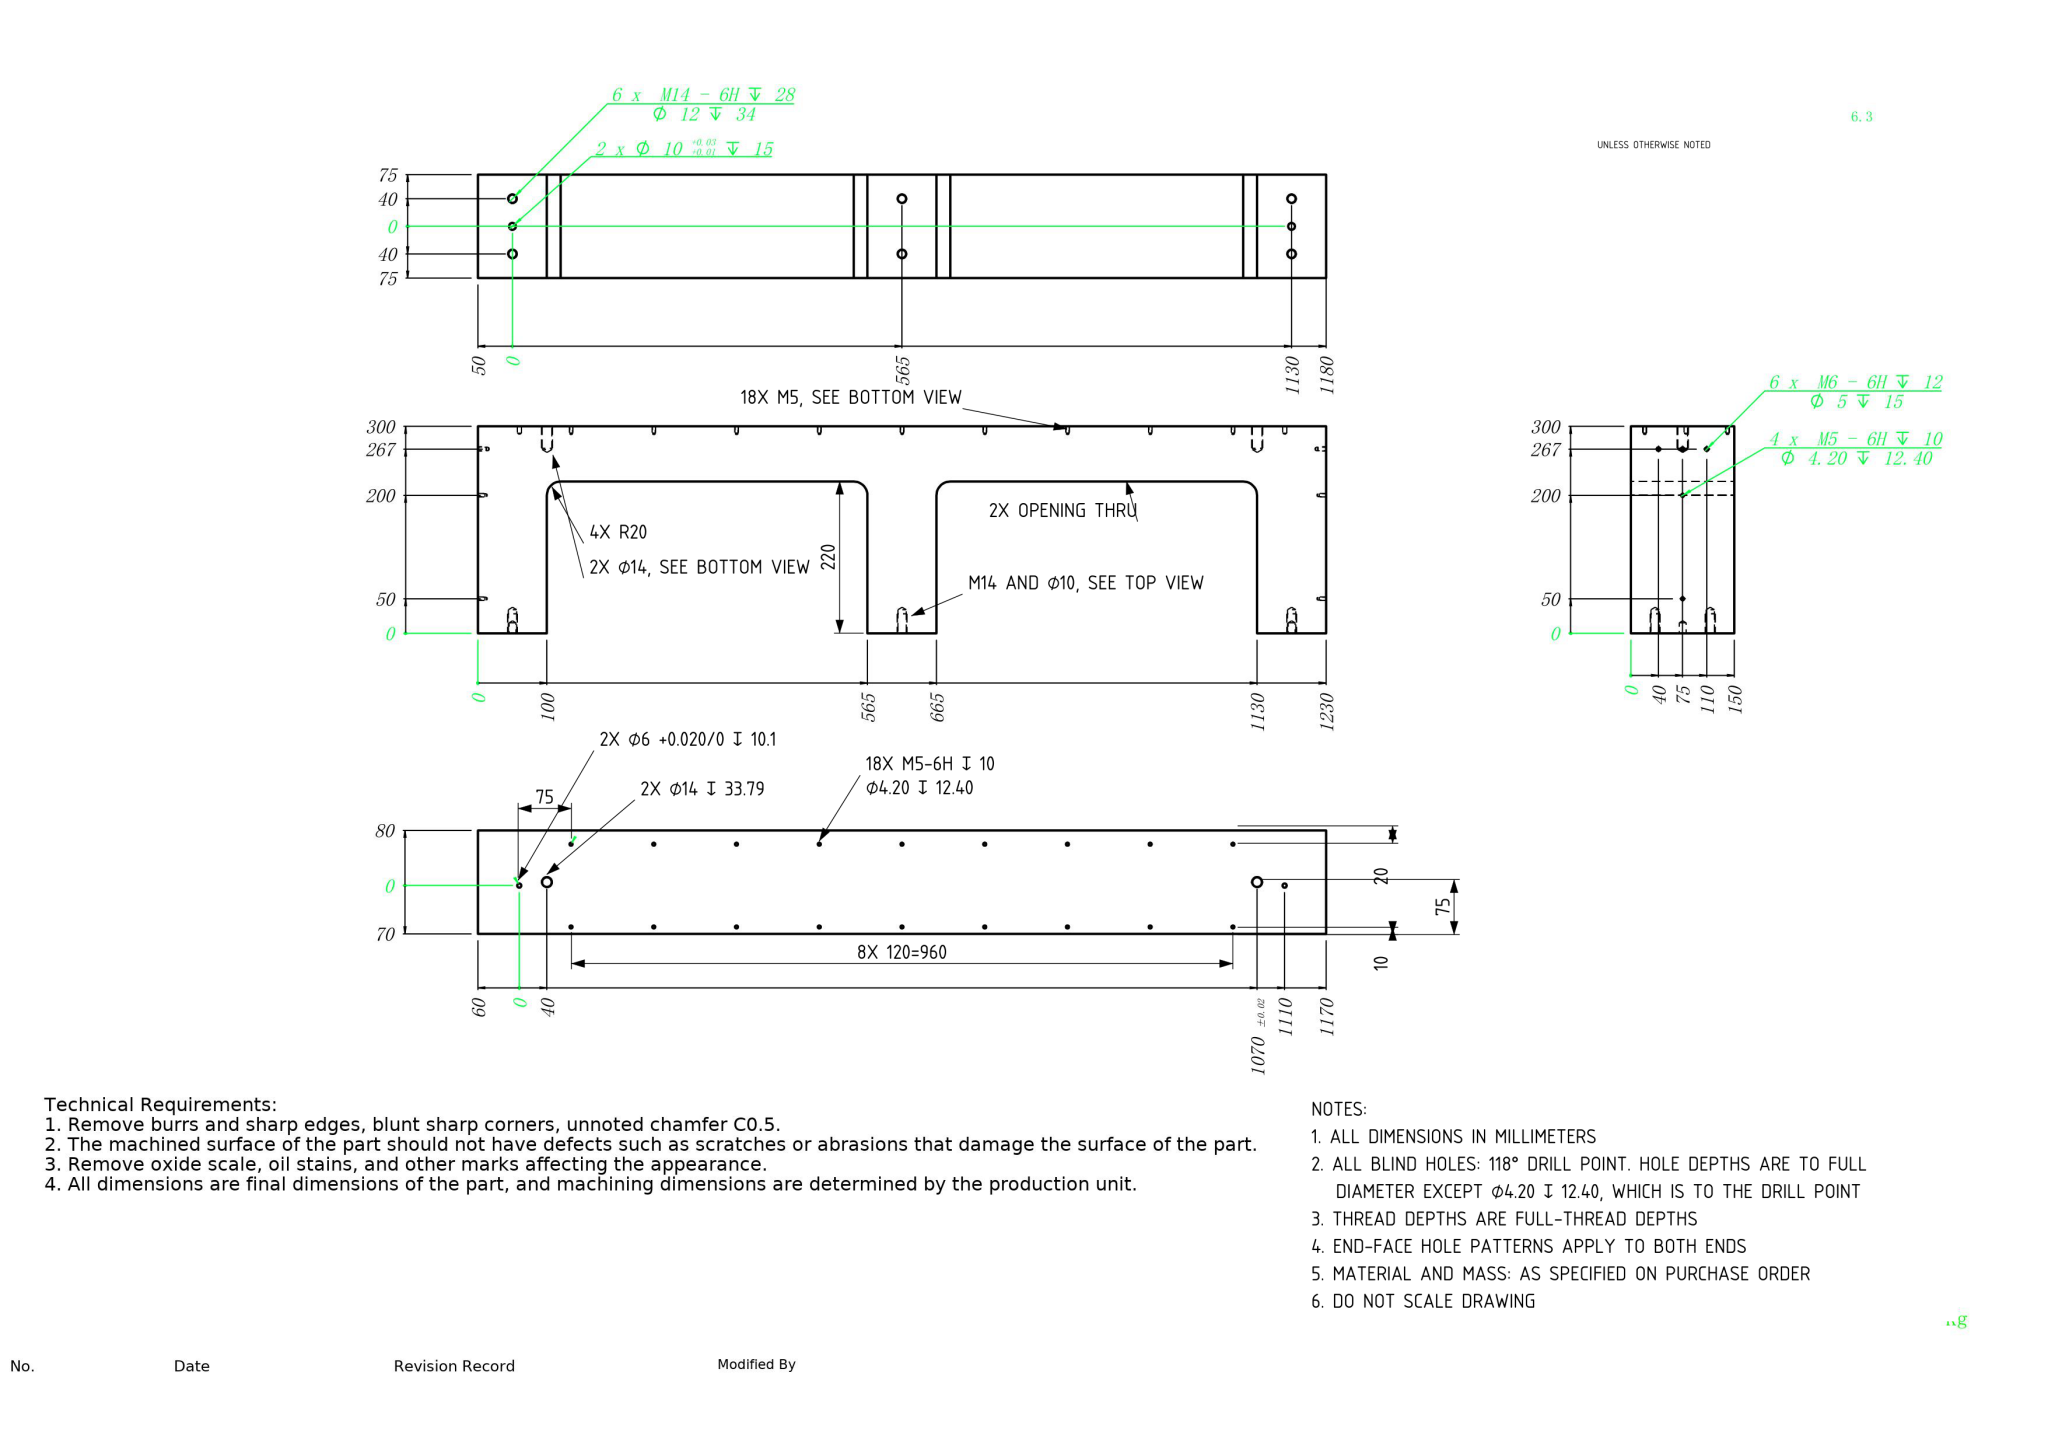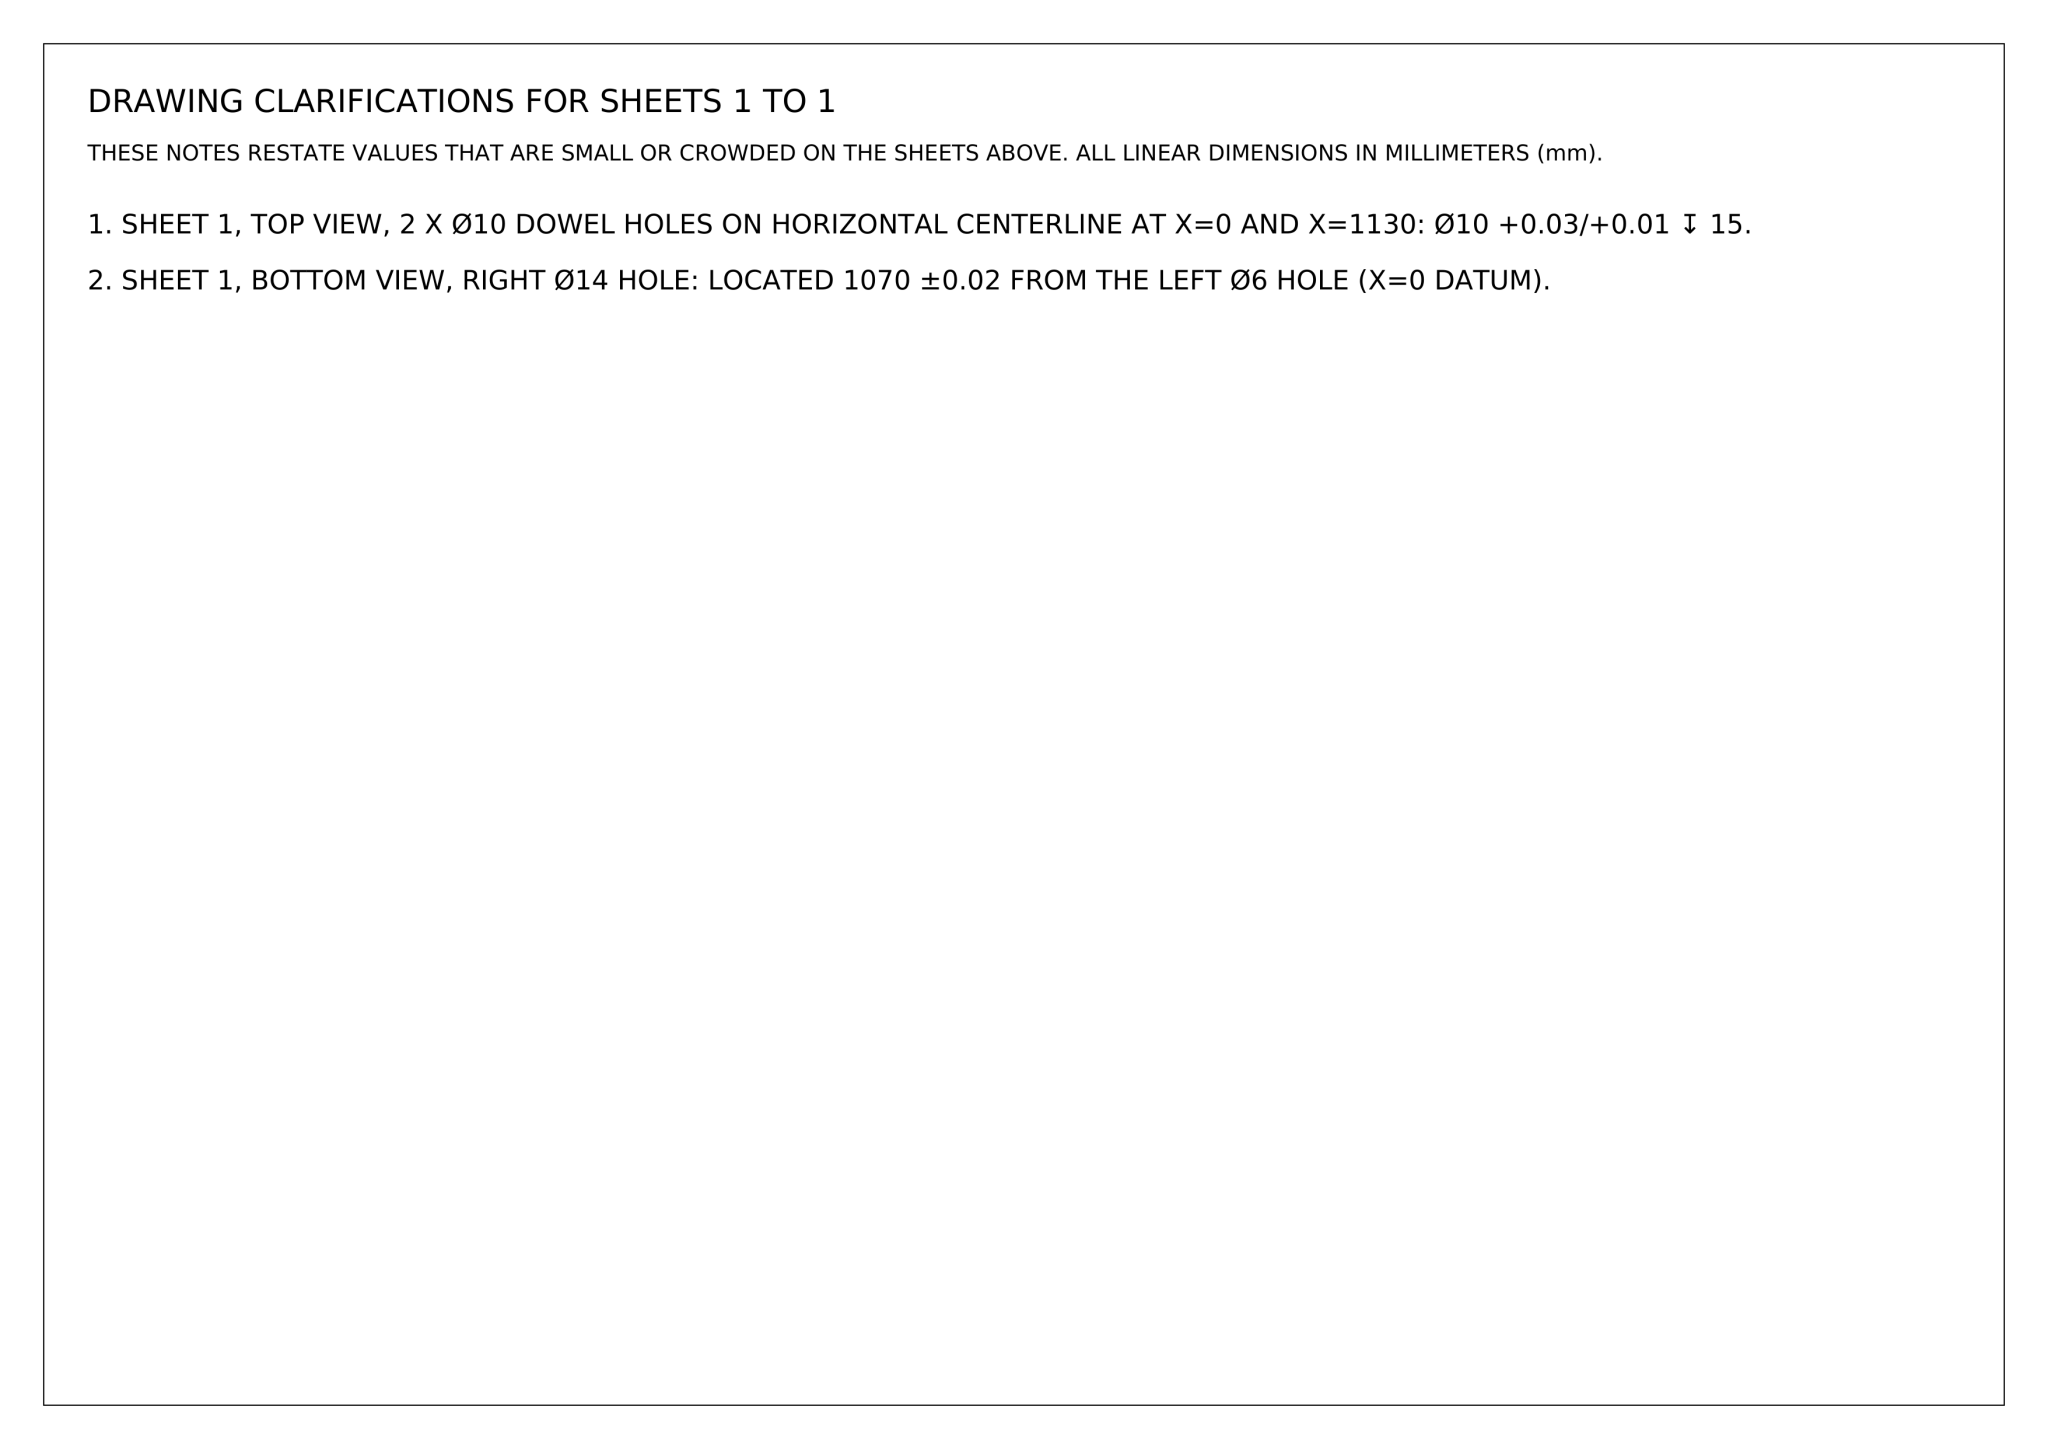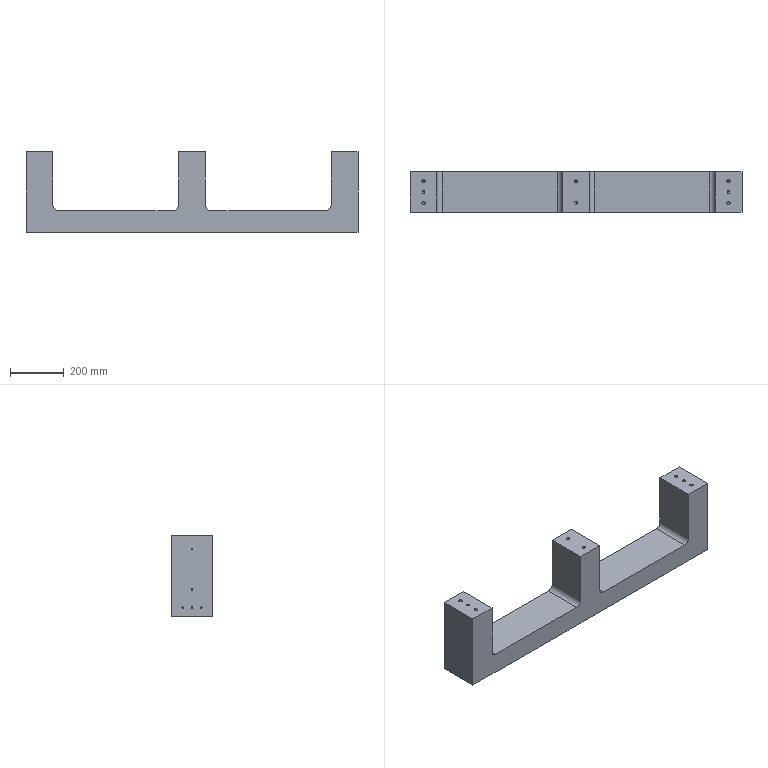Part | NX | mm | 1 solid | 178 faces | box 1230 x 150 x 300 mm | volume 24668243 mm3 | cylinder 84 | cone 80 | plane 14 | commonest cylinder face diameters 4.2 x44 5 x12 12 x12 6 x4 14 x4 10 x4 40 x4